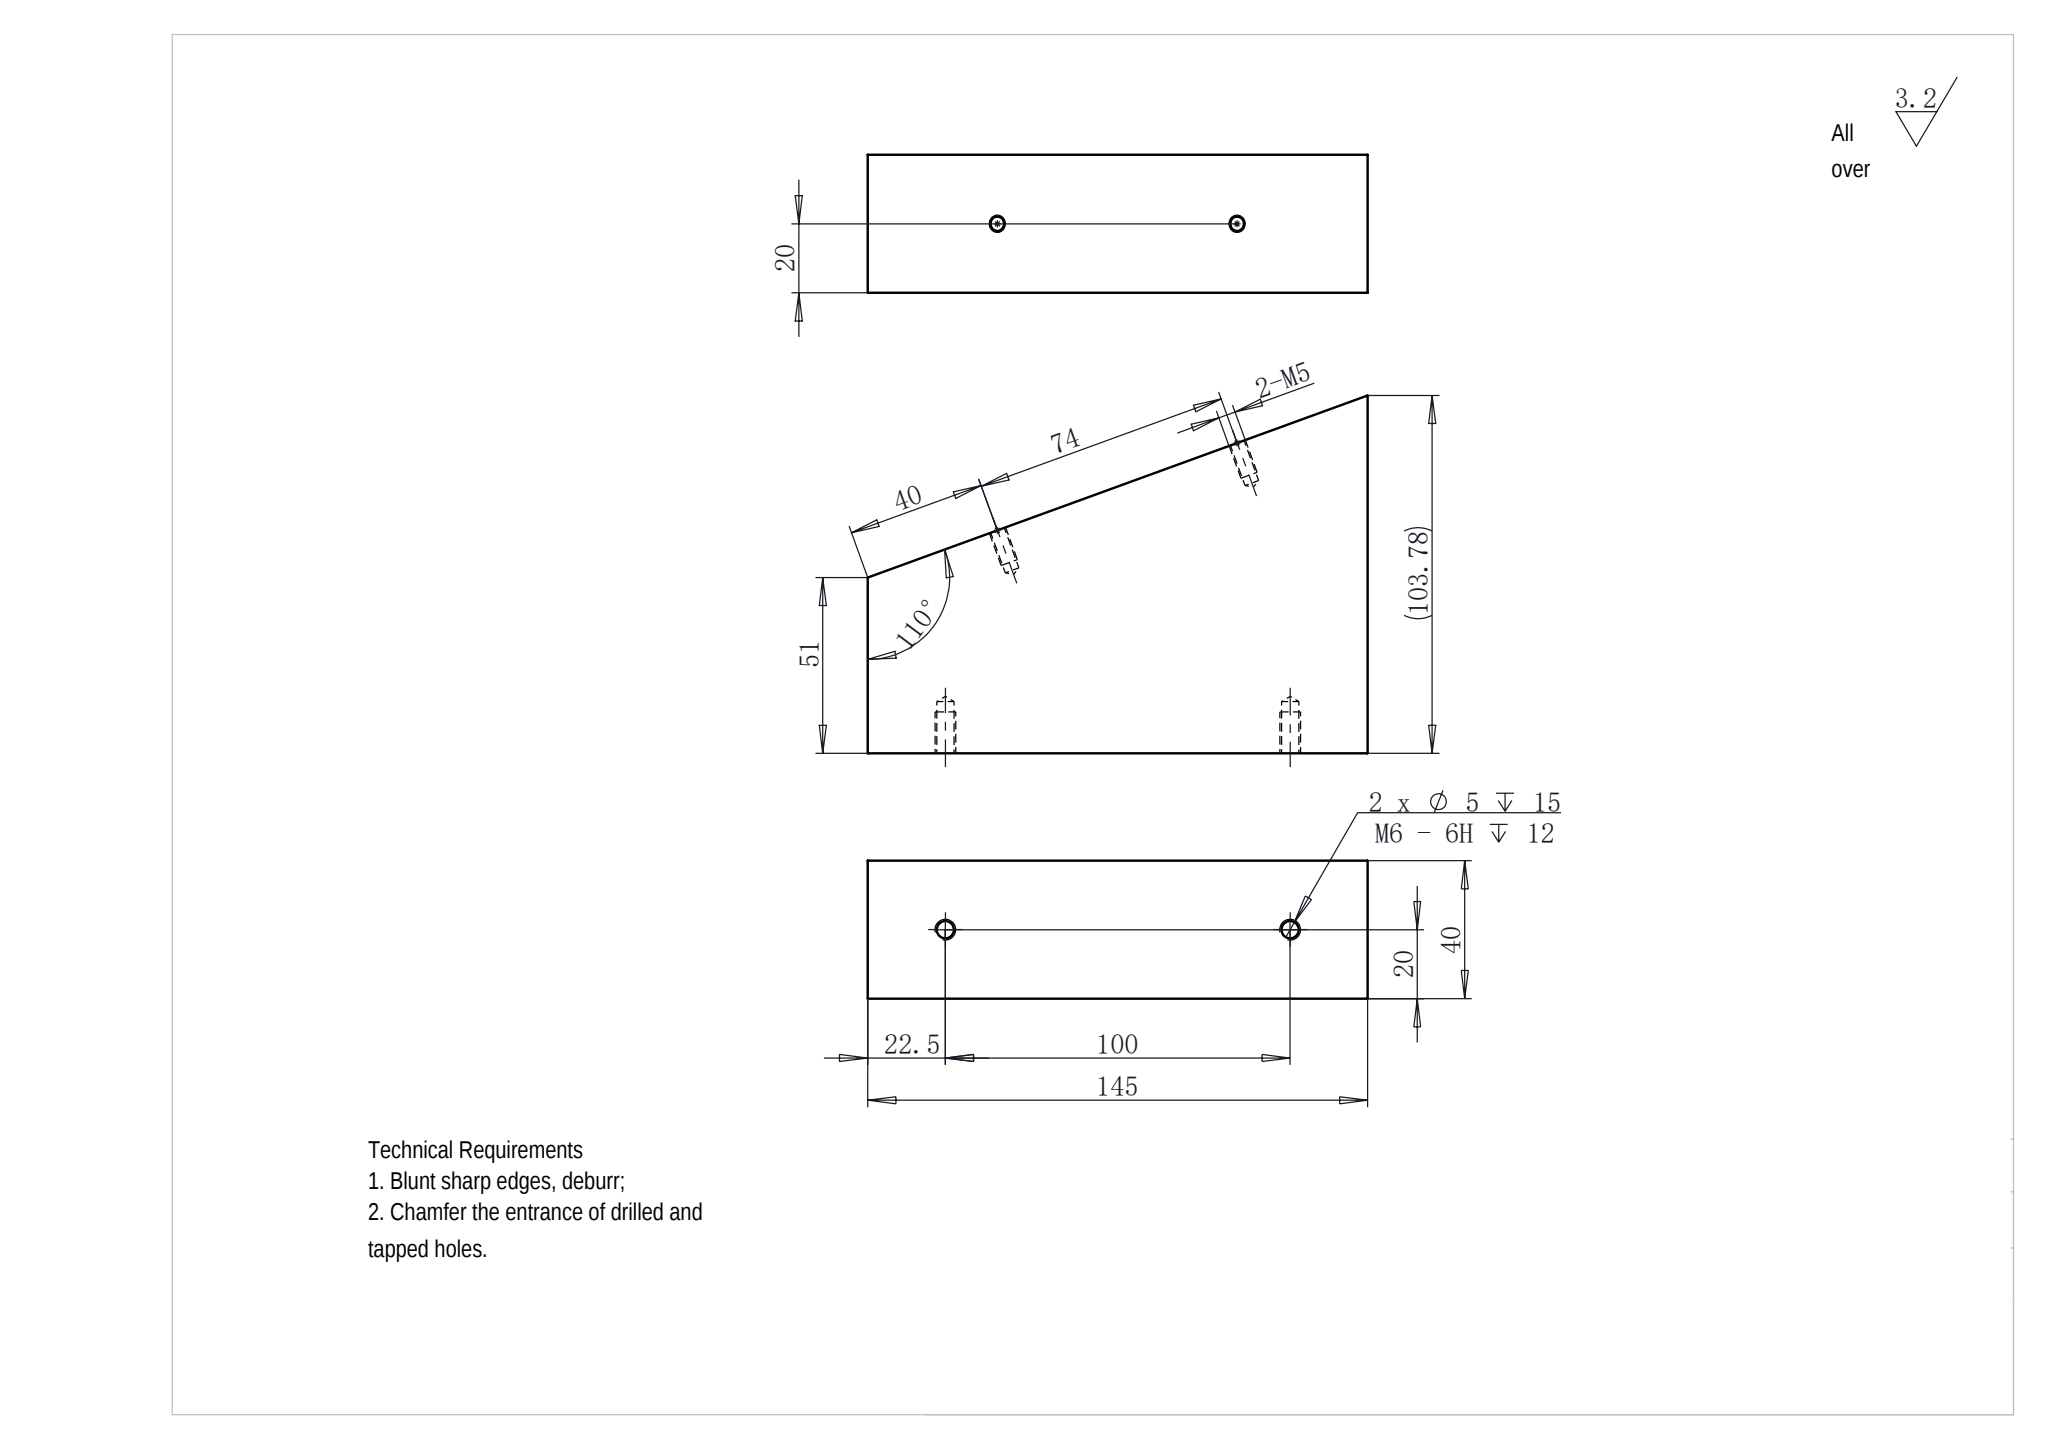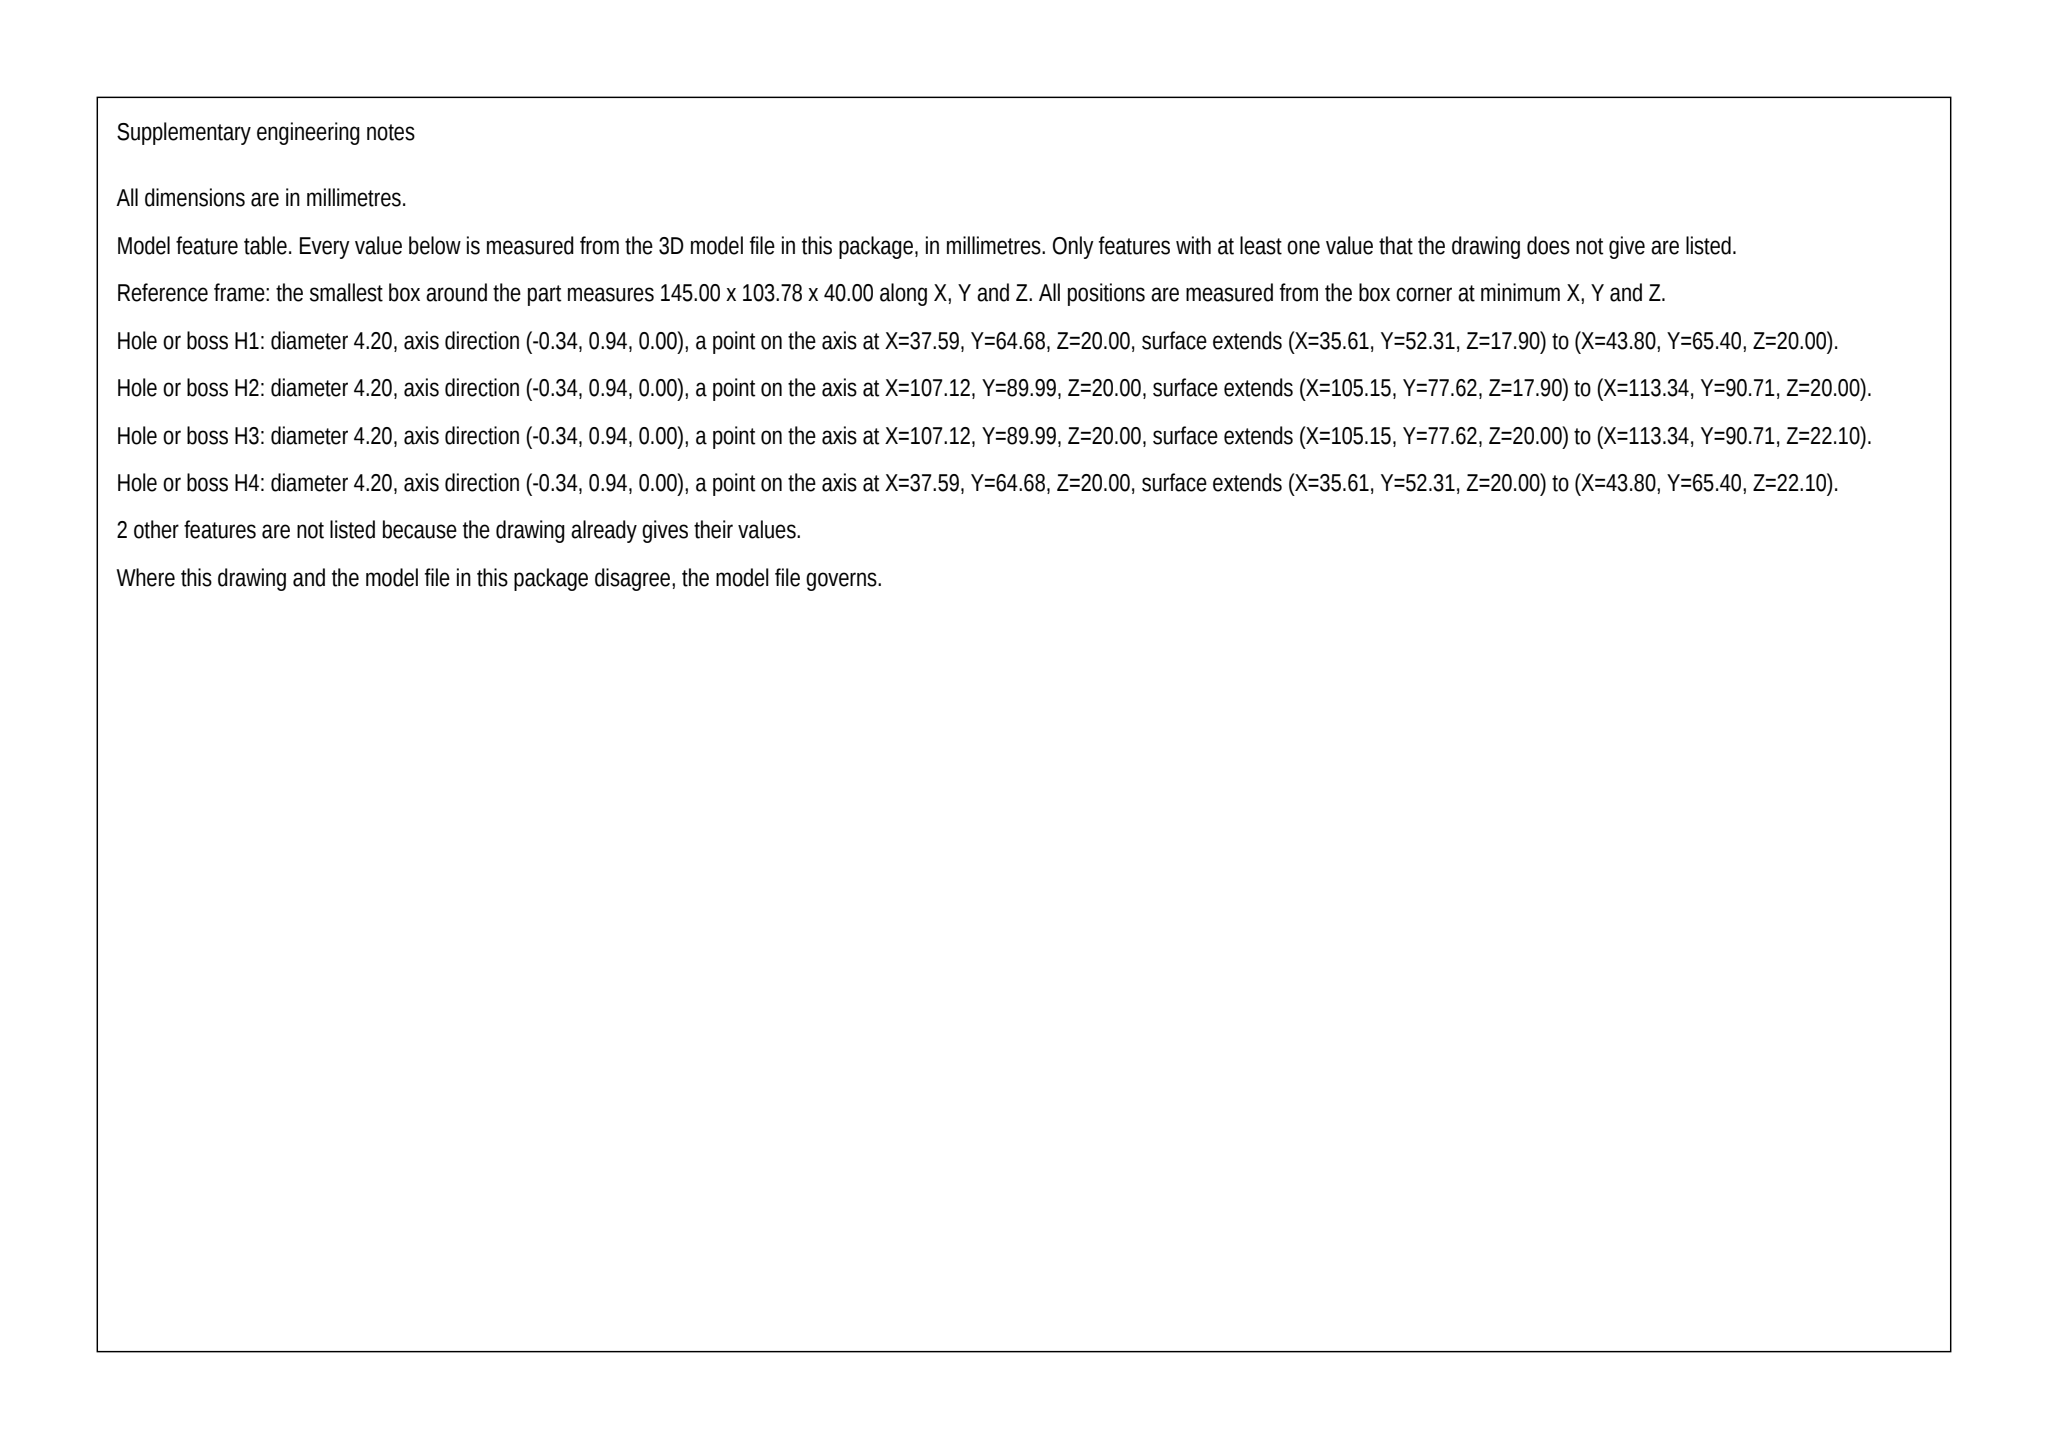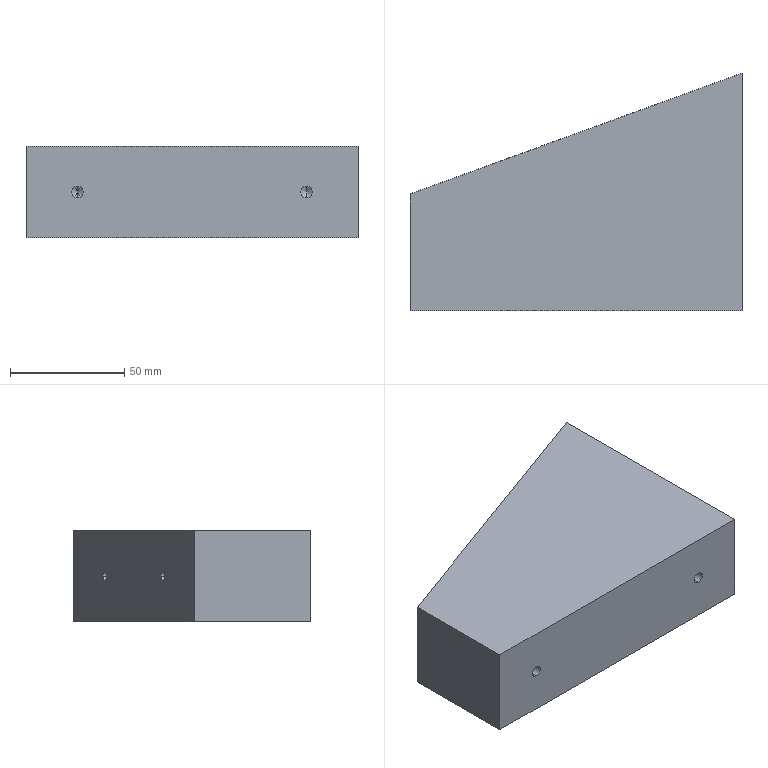Part | SolidWorks | mm | 1 solid | 22 faces | box 145 x 103.78 x 40 mm | volume 447886 mm3 | cylinder 8 | cone 8 | plane 6 | commonest cylinder face diameters 5 x4 4.2 x4
build123d program:
from build123d import *

# Parameters (mm, degrees)
BOSS_EXTRUDE1_DEPTH   = 40
M5_TAPPED_HOLE1_D     = 4.2
M5_TAPPED_HOLE1_DEPTH = 12.4
M5_TAPPED_HOLE1_TIP   = 1.262
M6_TAPPED_HOLE1_D     = 5
M6_TAPPED_HOLE1_DEPTH = 15
M6_TAPPED_HOLE1_TIP   = 1.502


with BuildPart() as part:
    # Sketch1 → Boss-Extrude1 (new body)
    with BuildSketch(Plane.XY):
        Polygon((0, 0), (0, 51), (145, 103.776), (145, 0), align=None)
    extrude(amount=-BOSS_EXTRUDE1_DEPTH)

    # M5 Tapped Hole1
    with Locations(Plane(origin=(-16.391, 45.034, 0), x_dir=(0.9397, 0.342, 0), z_dir=(-0.342, 0.9397, 0))):
        with Locations((57.443, 20), (131.443, 20)):
            Hole(M5_TAPPED_HOLE1_D / 2, depth=M5_TAPPED_HOLE1_DEPTH)
            with Locations((0, 0, -(M5_TAPPED_HOLE1_DEPTH + M5_TAPPED_HOLE1_TIP / 2))):  # 118° drill point
                Cone(0, M5_TAPPED_HOLE1_D / 2, M5_TAPPED_HOLE1_TIP, mode=Mode.SUBTRACT)

    # M6 Tapped Hole1
    with Locations(Plane(origin=(0, 0, 0), x_dir=(-1, 0, 0), z_dir=(0, -1, 0))):
        with Locations((-22.5, 20), (-122.5, 20)):
            Hole(M6_TAPPED_HOLE1_D / 2, depth=M6_TAPPED_HOLE1_DEPTH)
            with Locations((0, 0, -(M6_TAPPED_HOLE1_DEPTH + M6_TAPPED_HOLE1_TIP / 2))):  # 118° drill point
                Cone(0, M6_TAPPED_HOLE1_D / 2, M6_TAPPED_HOLE1_TIP, mode=Mode.SUBTRACT)


solid = part.part
STEP:
#1=CARTESIAN_POINT('',(22.5,15.,-17.5));
#2=VERTEX_POINT('',#1);
#3=CARTESIAN_POINT('',(22.5,15.,-22.5));
#4=VERTEX_POINT('',#3);
#5=CARTESIAN_POINT('',(22.5,15.,-20.));
#6=DIRECTION('',(0.,-1.,0.));
#7=DIRECTION('',(0.,0.,-1.));
#8=AXIS2_PLACEMENT_3D('',#5,#6,#7);
#9=CIRCLE('',#8,2.5);
#10=EDGE_CURVE('',#2,#4,#9,.T.);
#11=ORIENTED_EDGE('',*,*,#10,.F.);
#12=CARTESIAN_POINT('',(22.5,-0.,-17.5));
#13=VERTEX_POINT('',#12);
#14=CARTESIAN_POINT('',(22.5,0.,-17.5));
#15=DIRECTION('',(0.,-1.,0.));
#16=VECTOR('',#15,1000.);
#17=LINE('',#14,#16);
#18=EDGE_CURVE('',#2,#13,#17,.T.);
#19=ORIENTED_EDGE('',*,*,#18,.T.);
#20=CARTESIAN_POINT('',(22.5,-0.,-22.5));
#21=VERTEX_POINT('',#20);
#22=CARTESIAN_POINT('',(22.5,-0.,-20.));
#23=DIRECTION('',(0.,-1.,0.));
#24=DIRECTION('',(0.,0.,-1.));
#25=AXIS2_PLACEMENT_3D('',#22,#23,#24);
#26=CIRCLE('',#25,2.5);
#27=EDGE_CURVE('',#13,#21,#26,.T.);
#28=ORIENTED_EDGE('',*,*,#27,.T.);
#29=CARTESIAN_POINT('',(22.5,0.,-22.5));
#30=DIRECTION('',(0.,-1.,0.));
#31=VECTOR('',#30,1000.);
#32=LINE('',#29,#31);
#33=EDGE_CURVE('',#4,#21,#32,.T.);
#34=ORIENTED_EDGE('',*,*,#33,.F.);
#35=EDGE_LOOP('',(#11,#19,#28,#34));
#36=FACE_OUTER_BOUND('',#35,.T.);
#37=CARTESIAN_POINT('',(22.5,0.,-20.));
#38=DIRECTION('',(0.,-1.,0.));
#39=DIRECTION('',(0.,0.,-1.));
#40=AXIS2_PLACEMENT_3D('',#37,#38,#39);
#41=CYLINDRICAL_SURFACE('',#40,2.5);
#42=ADVANCED_FACE('',(#36),#41,.F.);
#43=CARTESIAN_POINT('',(22.5,16.502,-20.));
#44=VERTEX_POINT('',#43);
#45=CARTESIAN_POINT('',(22.5,15.,-22.5));
#46=DIRECTION('',(0.,-0.515,-0.8572));
#47=VECTOR('',#46,1000.);
#48=LINE('',#45,#47);
#49=EDGE_CURVE('',#44,#4,#48,.T.);
#50=ORIENTED_EDGE('',*,*,#49,.F.);
#51=CARTESIAN_POINT('',(22.5,15.,-17.5));
#52=DIRECTION('',(0.,-0.515,0.8572));
#53=VECTOR('',#52,1000.);
#54=LINE('',#51,#53);
#55=EDGE_CURVE('',#44,#2,#54,.T.);
#56=ORIENTED_EDGE('',*,*,#55,.T.);
#57=ORIENTED_EDGE('',*,*,#10,.T.);
#58=EDGE_LOOP('',(#50,#56,#57));
#59=FACE_OUTER_BOUND('',#58,.T.);
#60=CARTESIAN_POINT('',(22.5,15.,-20.));
#61=DIRECTION('',(0.,-1.,0.));
#62=DIRECTION('',(0.,0.,-1.));
#63=AXIS2_PLACEMENT_3D('',#60,#61,#62);
#64=CONICAL_SURFACE('',#63,2.5,1.03);
#65=ADVANCED_FACE('',(#59),#64,.F.);
#66=CARTESIAN_POINT('',(122.5,15.,-17.5));
#67=VERTEX_POINT('',#66);
#68=CARTESIAN_POINT('',(122.5,15.,-22.5));
#69=VERTEX_POINT('',#68);
#70=CARTESIAN_POINT('',(122.5,15.,-20.));
#71=DIRECTION('',(0.,-1.,0.));
#72=DIRECTION('',(0.,0.,-1.));
#73=AXIS2_PLACEMENT_3D('',#70,#71,#72);
#74=CIRCLE('',#73,2.5);
#75=EDGE_CURVE('',#67,#69,#74,.T.);
#76=ORIENTED_EDGE('',*,*,#75,.F.);
#77=CARTESIAN_POINT('',(122.5,0.,-17.5));
#78=VERTEX_POINT('',#77);
#79=CARTESIAN_POINT('',(122.5,0.,-17.5));
#80=DIRECTION('',(0.,-1.,0.));
#81=VECTOR('',#80,1000.);
#82=LINE('',#79,#81);
#83=EDGE_CURVE('',#67,#78,#82,.T.);
#84=ORIENTED_EDGE('',*,*,#83,.T.);
#85=CARTESIAN_POINT('',(122.5,0.,-22.5));
#86=VERTEX_POINT('',#85);
#87=CARTESIAN_POINT('',(122.5,0.,-20.));
#88=DIRECTION('',(0.,-1.,0.));
#89=DIRECTION('',(0.,0.,-1.));
#90=AXIS2_PLACEMENT_3D('',#87,#88,#89);
#91=CIRCLE('',#90,2.5);
#92=EDGE_CURVE('',#78,#86,#91,.T.);
#93=ORIENTED_EDGE('',*,*,#92,.T.);
#94=CARTESIAN_POINT('',(122.5,0.,-22.5));
#95=DIRECTION('',(0.,-1.,0.));
#96=VECTOR('',#95,1000.);
#97=LINE('',#94,#96);
#98=EDGE_CURVE('',#69,#86,#97,.T.);
#99=ORIENTED_EDGE('',*,*,#98,.F.);
#100=EDGE_LOOP('',(#76,#84,#93,#99));
#101=FACE_OUTER_BOUND('',#100,.T.);
#102=CARTESIAN_POINT('',(122.5,0.,-20.));
#103=DIRECTION('',(0.,-1.,0.));
#104=DIRECTION('',(0.,0.,-1.));
#105=AXIS2_PLACEMENT_3D('',#102,#103,#104);
#106=CYLINDRICAL_SURFACE('',#105,2.5);
#107=ADVANCED_FACE('',(#101),#106,.F.);
#108=CARTESIAN_POINT('',(122.5,16.502,-20.));
#109=VERTEX_POINT('',#108);
#110=CARTESIAN_POINT('',(122.5,15.,-22.5));
#111=DIRECTION('',(0.,-0.515,-0.8572));
#112=VECTOR('',#111,1000.);
#113=LINE('',#110,#112);
#114=EDGE_CURVE('',#109,#69,#113,.T.);
#115=ORIENTED_EDGE('',*,*,#114,.F.);
#116=CARTESIAN_POINT('',(122.5,15.,-17.5));
#117=DIRECTION('',(0.,-0.515,0.8572));
#118=VECTOR('',#117,1000.);
#119=LINE('',#116,#118);
#120=EDGE_CURVE('',#109,#67,#119,.T.);
#121=ORIENTED_EDGE('',*,*,#120,.T.);
#122=ORIENTED_EDGE('',*,*,#75,.T.);
#123=EDGE_LOOP('',(#115,#121,#122));
#124=FACE_OUTER_BOUND('',#123,.T.);
#125=CARTESIAN_POINT('',(122.5,15.,-20.));
#126=DIRECTION('',(0.,-1.,0.));
#127=DIRECTION('',(0.,0.,-1.));
#128=AXIS2_PLACEMENT_3D('',#125,#126,#127);
#129=CONICAL_SURFACE('',#128,2.5,1.03);
#130=ADVANCED_FACE('',(#124),#129,.F.);
#131=CARTESIAN_POINT('',(43.802,53.747,-20.));
#132=VERTEX_POINT('',#131);
#133=CARTESIAN_POINT('',(39.855,52.31,-20.));
#134=VERTEX_POINT('',#133);
#135=CARTESIAN_POINT('',(41.829,53.029,-20.));
#136=DIRECTION('',(-0.342,0.9397,0.));
#137=DIRECTION('',(-0.9397,-0.342,0.));
#138=AXIS2_PLACEMENT_3D('',#135,#136,#137);
#139=CIRCLE('',#138,2.1);
#140=EDGE_CURVE('',#132,#134,#139,.T.);
#141=ORIENTED_EDGE('',*,*,#140,.F.);
#142=CARTESIAN_POINT('',(39.561,65.399,-20.));
#143=VERTEX_POINT('',#142);
#144=CARTESIAN_POINT('',(39.561,65.399,-20.));
#145=DIRECTION('',(-0.342,0.9397,0.));
#146=VECTOR('',#145,1000.);
#147=LINE('',#144,#146);
#148=EDGE_CURVE('',#132,#143,#147,.T.);
#149=ORIENTED_EDGE('',*,*,#148,.T.);
#150=CARTESIAN_POINT('',(35.614,63.963,-20.));
#151=VERTEX_POINT('',#150);
#152=CARTESIAN_POINT('',(37.588,64.681,-20.));
#153=DIRECTION('',(-0.342,0.9397,0.));
#154=DIRECTION('',(-0.9397,-0.342,0.));
#155=AXIS2_PLACEMENT_3D('',#152,#153,#154);
#156=CIRCLE('',#155,2.1);
#157=EDGE_CURVE('',#143,#151,#156,.T.);
#158=ORIENTED_EDGE('',*,*,#157,.T.);
#159=CARTESIAN_POINT('',(35.614,63.963,-20.));
#160=DIRECTION('',(-0.342,0.9397,0.));
#161=VECTOR('',#160,1000.);
#162=LINE('',#159,#161);
#163=EDGE_CURVE('',#134,#151,#162,.T.);
#164=ORIENTED_EDGE('',*,*,#163,.F.);
#165=EDGE_LOOP('',(#141,#149,#158,#164));
#166=FACE_OUTER_BOUND('',#165,.T.);
#167=CARTESIAN_POINT('',(37.588,64.681,-20.));
#168=DIRECTION('',(-0.342,0.9397,0.));
#169=DIRECTION('',(-0.9397,-0.342,0.));
#170=AXIS2_PLACEMENT_3D('',#167,#168,#169);
#171=CYLINDRICAL_SURFACE('',#170,2.1);
#172=ADVANCED_FACE('',(#166),#171,.F.);
#173=CARTESIAN_POINT('',(42.26,51.843,-20.));
#174=VERTEX_POINT('',#173);
#175=CARTESIAN_POINT('',(39.855,52.31,-20.));
#176=DIRECTION('',(-0.9816,0.1908,0.));
#177=VECTOR('',#176,1000.);
#178=LINE('',#175,#177);
#179=EDGE_CURVE('',#174,#134,#178,.T.);
#180=ORIENTED_EDGE('',*,*,#179,.F.);
#181=CARTESIAN_POINT('',(43.802,53.747,-20.));
#182=DIRECTION('',(0.6293,0.7771,0.));
#183=VECTOR('',#182,1000.);
#184=LINE('',#181,#183);
#185=EDGE_CURVE('',#174,#132,#184,.T.);
#186=ORIENTED_EDGE('',*,*,#185,.T.);
#187=ORIENTED_EDGE('',*,*,#140,.T.);
#188=EDGE_LOOP('',(#180,#186,#187));
#189=FACE_OUTER_BOUND('',#188,.T.);
#190=CARTESIAN_POINT('',(41.829,53.029,-20.));
#191=DIRECTION('',(-0.342,0.9397,0.));
#192=DIRECTION('',(-0.9397,-0.342,0.));
#193=AXIS2_PLACEMENT_3D('',#190,#191,#192);
#194=CONICAL_SURFACE('',#193,2.1,1.03);
#195=ADVANCED_FACE('',(#189),#194,.F.);
#196=CARTESIAN_POINT('',(113.339,79.056,-20.));
#197=VERTEX_POINT('',#196);
#198=CARTESIAN_POINT('',(109.393,77.62,-20.));
#199=VERTEX_POINT('',#198);
#200=CARTESIAN_POINT('',(111.366,78.338,-20.));
#201=DIRECTION('',(-0.342,0.9397,0.));
#202=DIRECTION('',(-0.9397,-0.342,0.));
#203=AXIS2_PLACEMENT_3D('',#200,#201,#202);
#204=CIRCLE('',#203,2.1);
#205=EDGE_CURVE('',#197,#199,#204,.T.);
#206=ORIENTED_EDGE('',*,*,#205,.F.);
#207=CARTESIAN_POINT('',(109.098,90.709,-20.));
#208=VERTEX_POINT('',#207);
#209=CARTESIAN_POINT('',(109.098,90.709,-20.));
#210=DIRECTION('',(-0.342,0.9397,0.));
#211=VECTOR('',#210,1000.);
#212=LINE('',#209,#211);
#213=EDGE_CURVE('',#197,#208,#212,.T.);
#214=ORIENTED_EDGE('',*,*,#213,.T.);
#215=CARTESIAN_POINT('',(105.152,89.272,-20.));
#216=VERTEX_POINT('',#215);
#217=CARTESIAN_POINT('',(107.125,89.99,-20.));
#218=DIRECTION('',(-0.342,0.9397,0.));
#219=DIRECTION('',(-0.9397,-0.342,0.));
#220=AXIS2_PLACEMENT_3D('',#217,#218,#219);
#221=CIRCLE('',#220,2.1);
#222=EDGE_CURVE('',#208,#216,#221,.T.);
#223=ORIENTED_EDGE('',*,*,#222,.T.);
#224=CARTESIAN_POINT('',(105.152,89.272,-20.));
#225=DIRECTION('',(-0.342,0.9397,0.));
#226=VECTOR('',#225,1000.);
#227=LINE('',#224,#226);
#228=EDGE_CURVE('',#199,#216,#227,.T.);
#229=ORIENTED_EDGE('',*,*,#228,.F.);
#230=EDGE_LOOP('',(#206,#214,#223,#229));
#231=FACE_OUTER_BOUND('',#230,.T.);
#232=CARTESIAN_POINT('',(107.125,89.99,-20.));
#233=DIRECTION('',(-0.342,0.9397,0.));
#234=DIRECTION('',(-0.9397,-0.342,0.));
#235=AXIS2_PLACEMENT_3D('',#232,#233,#234);
#236=CYLINDRICAL_SURFACE('',#235,2.1);
#237=ADVANCED_FACE('',(#231),#236,.F.);
#238=CARTESIAN_POINT('',(111.798,77.152,-20.));
#239=VERTEX_POINT('',#238);
#240=CARTESIAN_POINT('',(109.393,77.62,-20.));
#241=DIRECTION('',(-0.9816,0.1908,0.));
#242=VECTOR('',#241,1000.);
#243=LINE('',#240,#242);
#244=EDGE_CURVE('',#239,#199,#243,.T.);
#245=ORIENTED_EDGE('',*,*,#244,.F.);
#246=CARTESIAN_POINT('',(113.339,79.056,-20.));
#247=DIRECTION('',(0.6293,0.7771,0.));
#248=VECTOR('',#247,1000.);
#249=LINE('',#246,#248);
#250=EDGE_CURVE('',#239,#197,#249,.T.);
#251=ORIENTED_EDGE('',*,*,#250,.T.);
#252=ORIENTED_EDGE('',*,*,#205,.T.);
#253=EDGE_LOOP('',(#245,#251,#252));
#254=FACE_OUTER_BOUND('',#253,.T.);
#255=CARTESIAN_POINT('',(111.366,78.338,-20.));
#256=DIRECTION('',(-0.342,0.9397,0.));
#257=DIRECTION('',(-0.9397,-0.342,0.));
#258=AXIS2_PLACEMENT_3D('',#255,#256,#257);
#259=CONICAL_SURFACE('',#258,2.1,1.03);
#260=ADVANCED_FACE('',(#254),#259,.F.);
#261=CARTESIAN_POINT('',(22.5,-0.,-20.));
#262=DIRECTION('',(0.,-1.,0.));
#263=DIRECTION('',(0.,0.,-1.));
#264=AXIS2_PLACEMENT_3D('',#261,#262,#263);
#265=CIRCLE('',#264,2.5);
#266=EDGE_CURVE('',#21,#13,#265,.T.);
#267=ORIENTED_EDGE('',*,*,#266,.F.);
#268=ORIENTED_EDGE('',*,*,#27,.F.);
#269=EDGE_LOOP('',(#267,#268));
#270=FACE_BOUND('',#269,.T.);
#271=CARTESIAN_POINT('',(122.5,0.,-20.));
#272=DIRECTION('',(0.,-1.,0.));
#273=DIRECTION('',(0.,0.,-1.));
#274=AXIS2_PLACEMENT_3D('',#271,#272,#273);
#275=CIRCLE('',#274,2.5);
#276=EDGE_CURVE('',#86,#78,#275,.T.);
#277=ORIENTED_EDGE('',*,*,#276,.F.);
#278=ORIENTED_EDGE('',*,*,#92,.F.);
#279=EDGE_LOOP('',(#277,#278));
#280=FACE_BOUND('',#279,.T.);
#281=CARTESIAN_POINT('',(0.,0.,0.));
#282=VERTEX_POINT('',#281);
#283=CARTESIAN_POINT('',(145.,0.,0.));
#284=VERTEX_POINT('',#283);
#285=CARTESIAN_POINT('',(145.,0.,0.));
#286=DIRECTION('',(1.,0.,0.));
#287=VECTOR('',#286,1000.);
#288=LINE('',#285,#287);
#289=EDGE_CURVE('',#282,#284,#288,.T.);
#290=ORIENTED_EDGE('',*,*,#289,.F.);
#291=CARTESIAN_POINT('',(0.,0.,-40.));
#292=VERTEX_POINT('',#291);
#293=CARTESIAN_POINT('',(0.,0.,-40.));
#294=DIRECTION('',(0.,0.,1.));
#295=VECTOR('',#294,1000.);
#296=LINE('',#293,#295);
#297=EDGE_CURVE('',#292,#282,#296,.T.);
#298=ORIENTED_EDGE('',*,*,#297,.F.);
#299=CARTESIAN_POINT('',(145.,0.,-40.));
#300=VERTEX_POINT('',#299);
#301=CARTESIAN_POINT('',(145.,0.,-40.));
#302=DIRECTION('',(1.,0.,0.));
#303=VECTOR('',#302,1000.);
#304=LINE('',#301,#303);
#305=EDGE_CURVE('',#292,#300,#304,.T.);
#306=ORIENTED_EDGE('',*,*,#305,.T.);
#307=CARTESIAN_POINT('',(145.,0.,-40.));
#308=DIRECTION('',(0.,0.,1.));
#309=VECTOR('',#308,1000.);
#310=LINE('',#307,#309);
#311=EDGE_CURVE('',#300,#284,#310,.T.);
#312=ORIENTED_EDGE('',*,*,#311,.T.);
#313=EDGE_LOOP('',(#290,#298,#306,#312));
#314=FACE_OUTER_BOUND('',#313,.T.);
#315=CARTESIAN_POINT('',(145.,0.,-40.));
#316=DIRECTION('',(0.,-1.,0.));
#317=DIRECTION('',(1.,0.,0.));
#318=AXIS2_PLACEMENT_3D('',#315,#316,#317);
#319=PLANE('',#318);
#320=ADVANCED_FACE('',(#270,#280,#314),#319,.T.);
#321=CARTESIAN_POINT('',(0.,51.,0.));
#322=VERTEX_POINT('',#321);
#323=CARTESIAN_POINT('',(0.,0.,0.));
#324=DIRECTION('',(0.,-1.,0.));
#325=VECTOR('',#324,1000.);
#326=LINE('',#323,#325);
#327=EDGE_CURVE('',#322,#282,#326,.T.);
#328=ORIENTED_EDGE('',*,*,#327,.F.);
#329=CARTESIAN_POINT('',(0.,51.,-40.));
#330=VERTEX_POINT('',#329);
#331=CARTESIAN_POINT('',(0.,51.,-40.));
#332=DIRECTION('',(0.,0.,1.));
#333=VECTOR('',#332,1000.);
#334=LINE('',#331,#333);
#335=EDGE_CURVE('',#330,#322,#334,.T.);
#336=ORIENTED_EDGE('',*,*,#335,.F.);
#337=CARTESIAN_POINT('',(0.,0.,-40.));
#338=DIRECTION('',(0.,-1.,0.));
#339=VECTOR('',#338,1000.);
#340=LINE('',#337,#339);
#341=EDGE_CURVE('',#330,#292,#340,.T.);
#342=ORIENTED_EDGE('',*,*,#341,.T.);
#343=ORIENTED_EDGE('',*,*,#297,.T.);
#344=EDGE_LOOP('',(#328,#336,#342,#343));
#345=FACE_OUTER_BOUND('',#344,.T.);
#346=CARTESIAN_POINT('',(0.,0.,-40.));
#347=DIRECTION('',(-1.,0.,0.));
#348=DIRECTION('',(0.,0.,1.));
#349=AXIS2_PLACEMENT_3D('',#346,#347,#348);
#350=PLANE('',#349);
#351=ADVANCED_FACE('',(#345),#350,.T.);
#352=CARTESIAN_POINT('',(37.588,64.681,-20.));
#353=DIRECTION('',(-0.342,0.9397,0.));
#354=DIRECTION('',(-0.9397,-0.342,0.));
#355=AXIS2_PLACEMENT_3D('',#352,#353,#354);
#356=CIRCLE('',#355,2.1);
#357=EDGE_CURVE('',#151,#143,#356,.T.);
#358=ORIENTED_EDGE('',*,*,#357,.F.);
#359=ORIENTED_EDGE('',*,*,#157,.F.);
#360=EDGE_LOOP('',(#358,#359));
#361=FACE_BOUND('',#360,.T.);
#362=CARTESIAN_POINT('',(107.125,89.99,-20.));
#363=DIRECTION('',(-0.342,0.9397,0.));
#364=DIRECTION('',(-0.9397,-0.342,0.));
#365=AXIS2_PLACEMENT_3D('',#362,#363,#364);
#366=CIRCLE('',#365,2.1);
#367=EDGE_CURVE('',#216,#208,#366,.T.);
#368=ORIENTED_EDGE('',*,*,#367,.F.);
#369=ORIENTED_EDGE('',*,*,#222,.F.);
#370=EDGE_LOOP('',(#368,#369));
#371=FACE_BOUND('',#370,.T.);
#372=CARTESIAN_POINT('',(145.,103.776,0.));
#373=VERTEX_POINT('',#372);
#374=CARTESIAN_POINT('',(0.,51.,0.));
#375=DIRECTION('',(-0.9397,-0.342,0.));
#376=VECTOR('',#375,1000.);
#377=LINE('',#374,#376);
#378=EDGE_CURVE('',#373,#322,#377,.T.);
#379=ORIENTED_EDGE('',*,*,#378,.F.);
#380=CARTESIAN_POINT('',(145.,103.776,-40.));
#381=VERTEX_POINT('',#380);
#382=CARTESIAN_POINT('',(145.,103.776,-40.));
#383=DIRECTION('',(0.,0.,1.));
#384=VECTOR('',#383,1000.);
#385=LINE('',#382,#384);
#386=EDGE_CURVE('',#381,#373,#385,.T.);
#387=ORIENTED_EDGE('',*,*,#386,.F.);
#388=CARTESIAN_POINT('',(0.,51.,-40.));
#389=DIRECTION('',(-0.9397,-0.342,0.));
#390=VECTOR('',#389,1000.);
#391=LINE('',#388,#390);
#392=EDGE_CURVE('',#381,#330,#391,.T.);
#393=ORIENTED_EDGE('',*,*,#392,.T.);
#394=ORIENTED_EDGE('',*,*,#335,.T.);
#395=EDGE_LOOP('',(#379,#387,#393,#394));
#396=FACE_OUTER_BOUND('',#395,.T.);
#397=CARTESIAN_POINT('',(0.,51.,-40.));
#398=DIRECTION('',(-0.342,0.9397,0.));
#399=DIRECTION('',(-0.9397,-0.342,0.));
#400=AXIS2_PLACEMENT_3D('',#397,#398,#399);
#401=PLANE('',#400);
#402=ADVANCED_FACE('',(#361,#371,#396),#401,.T.);
#403=CARTESIAN_POINT('',(145.,103.776,0.));
#404=DIRECTION('',(0.,1.,0.));
#405=VECTOR('',#404,1000.);
#406=LINE('',#403,#405);
#407=EDGE_CURVE('',#284,#373,#406,.T.);
#408=ORIENTED_EDGE('',*,*,#407,.F.);
#409=ORIENTED_EDGE('',*,*,#311,.F.);
#410=CARTESIAN_POINT('',(145.,103.776,-40.));
#411=DIRECTION('',(0.,1.,0.));
#412=VECTOR('',#411,1000.);
#413=LINE('',#410,#412);
#414=EDGE_CURVE('',#300,#381,#413,.T.);
#415=ORIENTED_EDGE('',*,*,#414,.T.);
#416=ORIENTED_EDGE('',*,*,#386,.T.);
#417=EDGE_LOOP('',(#408,#409,#415,#416));
#418=FACE_OUTER_BOUND('',#417,.T.);
#419=CARTESIAN_POINT('',(145.,103.776,-40.));
#420=DIRECTION('',(1.,0.,0.));
#421=DIRECTION('',(0.,0.,-1.));
#422=AXIS2_PLACEMENT_3D('',#419,#420,#421);
#423=PLANE('',#422);
#424=ADVANCED_FACE('',(#418),#423,.T.);
#425=ORIENTED_EDGE('',*,*,#305,.F.);
#426=ORIENTED_EDGE('',*,*,#341,.F.);
#427=ORIENTED_EDGE('',*,*,#392,.F.);
#428=ORIENTED_EDGE('',*,*,#414,.F.);
#429=EDGE_LOOP('',(#425,#426,#427,#428));
#430=FACE_OUTER_BOUND('',#429,.T.);
#431=CARTESIAN_POINT('',(0.,0.,-40.));
#432=DIRECTION('',(0.,0.,-1.));
#433=DIRECTION('',(-1.,0.,0.));
#434=AXIS2_PLACEMENT_3D('',#431,#432,#433);
#435=PLANE('',#434);
#436=ADVANCED_FACE('',(#430),#435,.T.);
#437=ORIENTED_EDGE('',*,*,#289,.T.);
#438=ORIENTED_EDGE('',*,*,#407,.T.);
#439=ORIENTED_EDGE('',*,*,#378,.T.);
#440=ORIENTED_EDGE('',*,*,#327,.T.);
#441=EDGE_LOOP('',(#437,#438,#439,#440));
#442=FACE_OUTER_BOUND('',#441,.T.);
#443=CARTESIAN_POINT('',(0.,0.,0.));
#444=DIRECTION('',(0.,0.,-1.));
#445=DIRECTION('',(-1.,0.,0.));
#446=AXIS2_PLACEMENT_3D('',#443,#444,#445);
#447=PLANE('',#446);
#448=ADVANCED_FACE('',(#442),#447,.F.);
#449=ORIENTED_EDGE('',*,*,#250,.F.);
#450=ORIENTED_EDGE('',*,*,#244,.T.);
#451=CARTESIAN_POINT('',(111.366,78.338,-20.));
#452=DIRECTION('',(-0.342,0.9397,0.));
#453=DIRECTION('',(-0.9397,-0.342,0.));
#454=AXIS2_PLACEMENT_3D('',#451,#452,#453);
#455=CIRCLE('',#454,2.1);
#456=EDGE_CURVE('',#199,#197,#455,.T.);
#457=ORIENTED_EDGE('',*,*,#456,.T.);
#458=EDGE_LOOP('',(#449,#450,#457));
#459=FACE_OUTER_BOUND('',#458,.T.);
#460=CARTESIAN_POINT('',(111.366,78.338,-20.));
#461=DIRECTION('',(-0.342,0.9397,0.));
#462=DIRECTION('',(-0.9397,-0.342,0.));
#463=AXIS2_PLACEMENT_3D('',#460,#461,#462);
#464=CONICAL_SURFACE('',#463,2.1,1.03);
#465=ADVANCED_FACE('',(#459),#464,.F.);
#466=ORIENTED_EDGE('',*,*,#213,.F.);
#467=ORIENTED_EDGE('',*,*,#456,.F.);
#468=ORIENTED_EDGE('',*,*,#228,.T.);
#469=ORIENTED_EDGE('',*,*,#367,.T.);
#470=EDGE_LOOP('',(#466,#467,#468,#469));
#471=FACE_OUTER_BOUND('',#470,.T.);
#472=CARTESIAN_POINT('',(107.125,89.99,-20.));
#473=DIRECTION('',(-0.342,0.9397,0.));
#474=DIRECTION('',(-0.9397,-0.342,0.));
#475=AXIS2_PLACEMENT_3D('',#472,#473,#474);
#476=CYLINDRICAL_SURFACE('',#475,2.1);
#477=ADVANCED_FACE('',(#471),#476,.F.);
#478=ORIENTED_EDGE('',*,*,#185,.F.);
#479=ORIENTED_EDGE('',*,*,#179,.T.);
#480=CARTESIAN_POINT('',(41.829,53.029,-20.));
#481=DIRECTION('',(-0.342,0.9397,0.));
#482=DIRECTION('',(-0.9397,-0.342,0.));
#483=AXIS2_PLACEMENT_3D('',#480,#481,#482);
#484=CIRCLE('',#483,2.1);
#485=EDGE_CURVE('',#134,#132,#484,.T.);
#486=ORIENTED_EDGE('',*,*,#485,.T.);
#487=EDGE_LOOP('',(#478,#479,#486));
#488=FACE_OUTER_BOUND('',#487,.T.);
#489=CARTESIAN_POINT('',(41.829,53.029,-20.));
#490=DIRECTION('',(-0.342,0.9397,0.));
#491=DIRECTION('',(-0.9397,-0.342,0.));
#492=AXIS2_PLACEMENT_3D('',#489,#490,#491);
#493=CONICAL_SURFACE('',#492,2.1,1.03);
#494=ADVANCED_FACE('',(#488),#493,.F.);
#495=ORIENTED_EDGE('',*,*,#148,.F.);
#496=ORIENTED_EDGE('',*,*,#485,.F.);
#497=ORIENTED_EDGE('',*,*,#163,.T.);
#498=ORIENTED_EDGE('',*,*,#357,.T.);
#499=EDGE_LOOP('',(#495,#496,#497,#498));
#500=FACE_OUTER_BOUND('',#499,.T.);
#501=CARTESIAN_POINT('',(37.588,64.681,-20.));
#502=DIRECTION('',(-0.342,0.9397,0.));
#503=DIRECTION('',(-0.9397,-0.342,0.));
#504=AXIS2_PLACEMENT_3D('',#501,#502,#503);
#505=CYLINDRICAL_SURFACE('',#504,2.1);
#506=ADVANCED_FACE('',(#500),#505,.F.);
#507=ORIENTED_EDGE('',*,*,#120,.F.);
#508=ORIENTED_EDGE('',*,*,#114,.T.);
#509=CARTESIAN_POINT('',(122.5,15.,-20.));
#510=DIRECTION('',(0.,-1.,0.));
#511=DIRECTION('',(0.,0.,-1.));
#512=AXIS2_PLACEMENT_3D('',#509,#510,#511);
#513=CIRCLE('',#512,2.5);
#514=EDGE_CURVE('',#69,#67,#513,.T.);
#515=ORIENTED_EDGE('',*,*,#514,.T.);
#516=EDGE_LOOP('',(#507,#508,#515));
#517=FACE_OUTER_BOUND('',#516,.T.);
#518=CARTESIAN_POINT('',(122.5,15.,-20.));
#519=DIRECTION('',(0.,-1.,0.));
#520=DIRECTION('',(0.,0.,-1.));
#521=AXIS2_PLACEMENT_3D('',#518,#519,#520);
#522=CONICAL_SURFACE('',#521,2.5,1.03);
#523=ADVANCED_FACE('',(#517),#522,.F.);
#524=ORIENTED_EDGE('',*,*,#83,.F.);
#525=ORIENTED_EDGE('',*,*,#514,.F.);
#526=ORIENTED_EDGE('',*,*,#98,.T.);
#527=ORIENTED_EDGE('',*,*,#276,.T.);
#528=EDGE_LOOP('',(#524,#525,#526,#527));
#529=FACE_OUTER_BOUND('',#528,.T.);
#530=CARTESIAN_POINT('',(122.5,0.,-20.));
#531=DIRECTION('',(0.,-1.,0.));
#532=DIRECTION('',(0.,0.,-1.));
#533=AXIS2_PLACEMENT_3D('',#530,#531,#532);
#534=CYLINDRICAL_SURFACE('',#533,2.5);
#535=ADVANCED_FACE('',(#529),#534,.F.);
#536=ORIENTED_EDGE('',*,*,#55,.F.);
#537=ORIENTED_EDGE('',*,*,#49,.T.);
#538=CARTESIAN_POINT('',(22.5,15.,-20.));
#539=DIRECTION('',(0.,-1.,0.));
#540=DIRECTION('',(0.,0.,-1.));
#541=AXIS2_PLACEMENT_3D('',#538,#539,#540);
#542=CIRCLE('',#541,2.5);
#543=EDGE_CURVE('',#4,#2,#542,.T.);
#544=ORIENTED_EDGE('',*,*,#543,.T.);
#545=EDGE_LOOP('',(#536,#537,#544));
#546=FACE_OUTER_BOUND('',#545,.T.);
#547=CARTESIAN_POINT('',(22.5,15.,-20.));
#548=DIRECTION('',(0.,-1.,0.));
#549=DIRECTION('',(0.,0.,-1.));
#550=AXIS2_PLACEMENT_3D('',#547,#548,#549);
#551=CONICAL_SURFACE('',#550,2.5,1.03);
#552=ADVANCED_FACE('',(#546),#551,.F.);
#553=ORIENTED_EDGE('',*,*,#18,.F.);
#554=ORIENTED_EDGE('',*,*,#543,.F.);
#555=ORIENTED_EDGE('',*,*,#33,.T.);
#556=ORIENTED_EDGE('',*,*,#266,.T.);
#557=EDGE_LOOP('',(#553,#554,#555,#556));
#558=FACE_OUTER_BOUND('',#557,.T.);
#559=CARTESIAN_POINT('',(22.5,0.,-20.));
#560=DIRECTION('',(0.,-1.,0.));
#561=DIRECTION('',(0.,0.,-1.));
#562=AXIS2_PLACEMENT_3D('',#559,#560,#561);
#563=CYLINDRICAL_SURFACE('',#562,2.5);
#564=ADVANCED_FACE('',(#558),#563,.F.);
#565=CLOSED_SHELL('',(#42,#65,#107,#130,#172,#195,#237,#260,#320,#351,#402,#424,#436,#448,#465,#477,#494,#506,#523,#535,#552,#564));
#566=MANIFOLD_SOLID_BREP('',#565);
#567=CARTESIAN_POINT('',(0.,0.,0.));
#568=DIRECTION('',(0.,0.,1.));
#569=DIRECTION('',(1.,0.,0.));
#570=AXIS2_PLACEMENT_3D('',#567,#568,#569);
#571=(LENGTH_UNIT()NAMED_UNIT(*)SI_UNIT(.MILLI.,.METRE.));
#572=UNCERTAINTY_MEASURE_WITH_UNIT(LENGTH_MEASURE(0.00001),#571,'','');
#573=(NAMED_UNIT(*)PLANE_ANGLE_UNIT()SI_UNIT($,.RADIAN.));
#574=(NAMED_UNIT(*)SI_UNIT($,.STERADIAN.)SOLID_ANGLE_UNIT());
#575=(GEOMETRIC_REPRESENTATION_CONTEXT(3)GLOBAL_UNCERTAINTY_ASSIGNED_CONTEXT((#572))GLOBAL_UNIT_ASSIGNED_CONTEXT((#571,#573,#574))REPRESENTATION_CONTEXT('',''));
#576=ADVANCED_BREP_SHAPE_REPRESENTATION('',(#566,#570),#575);